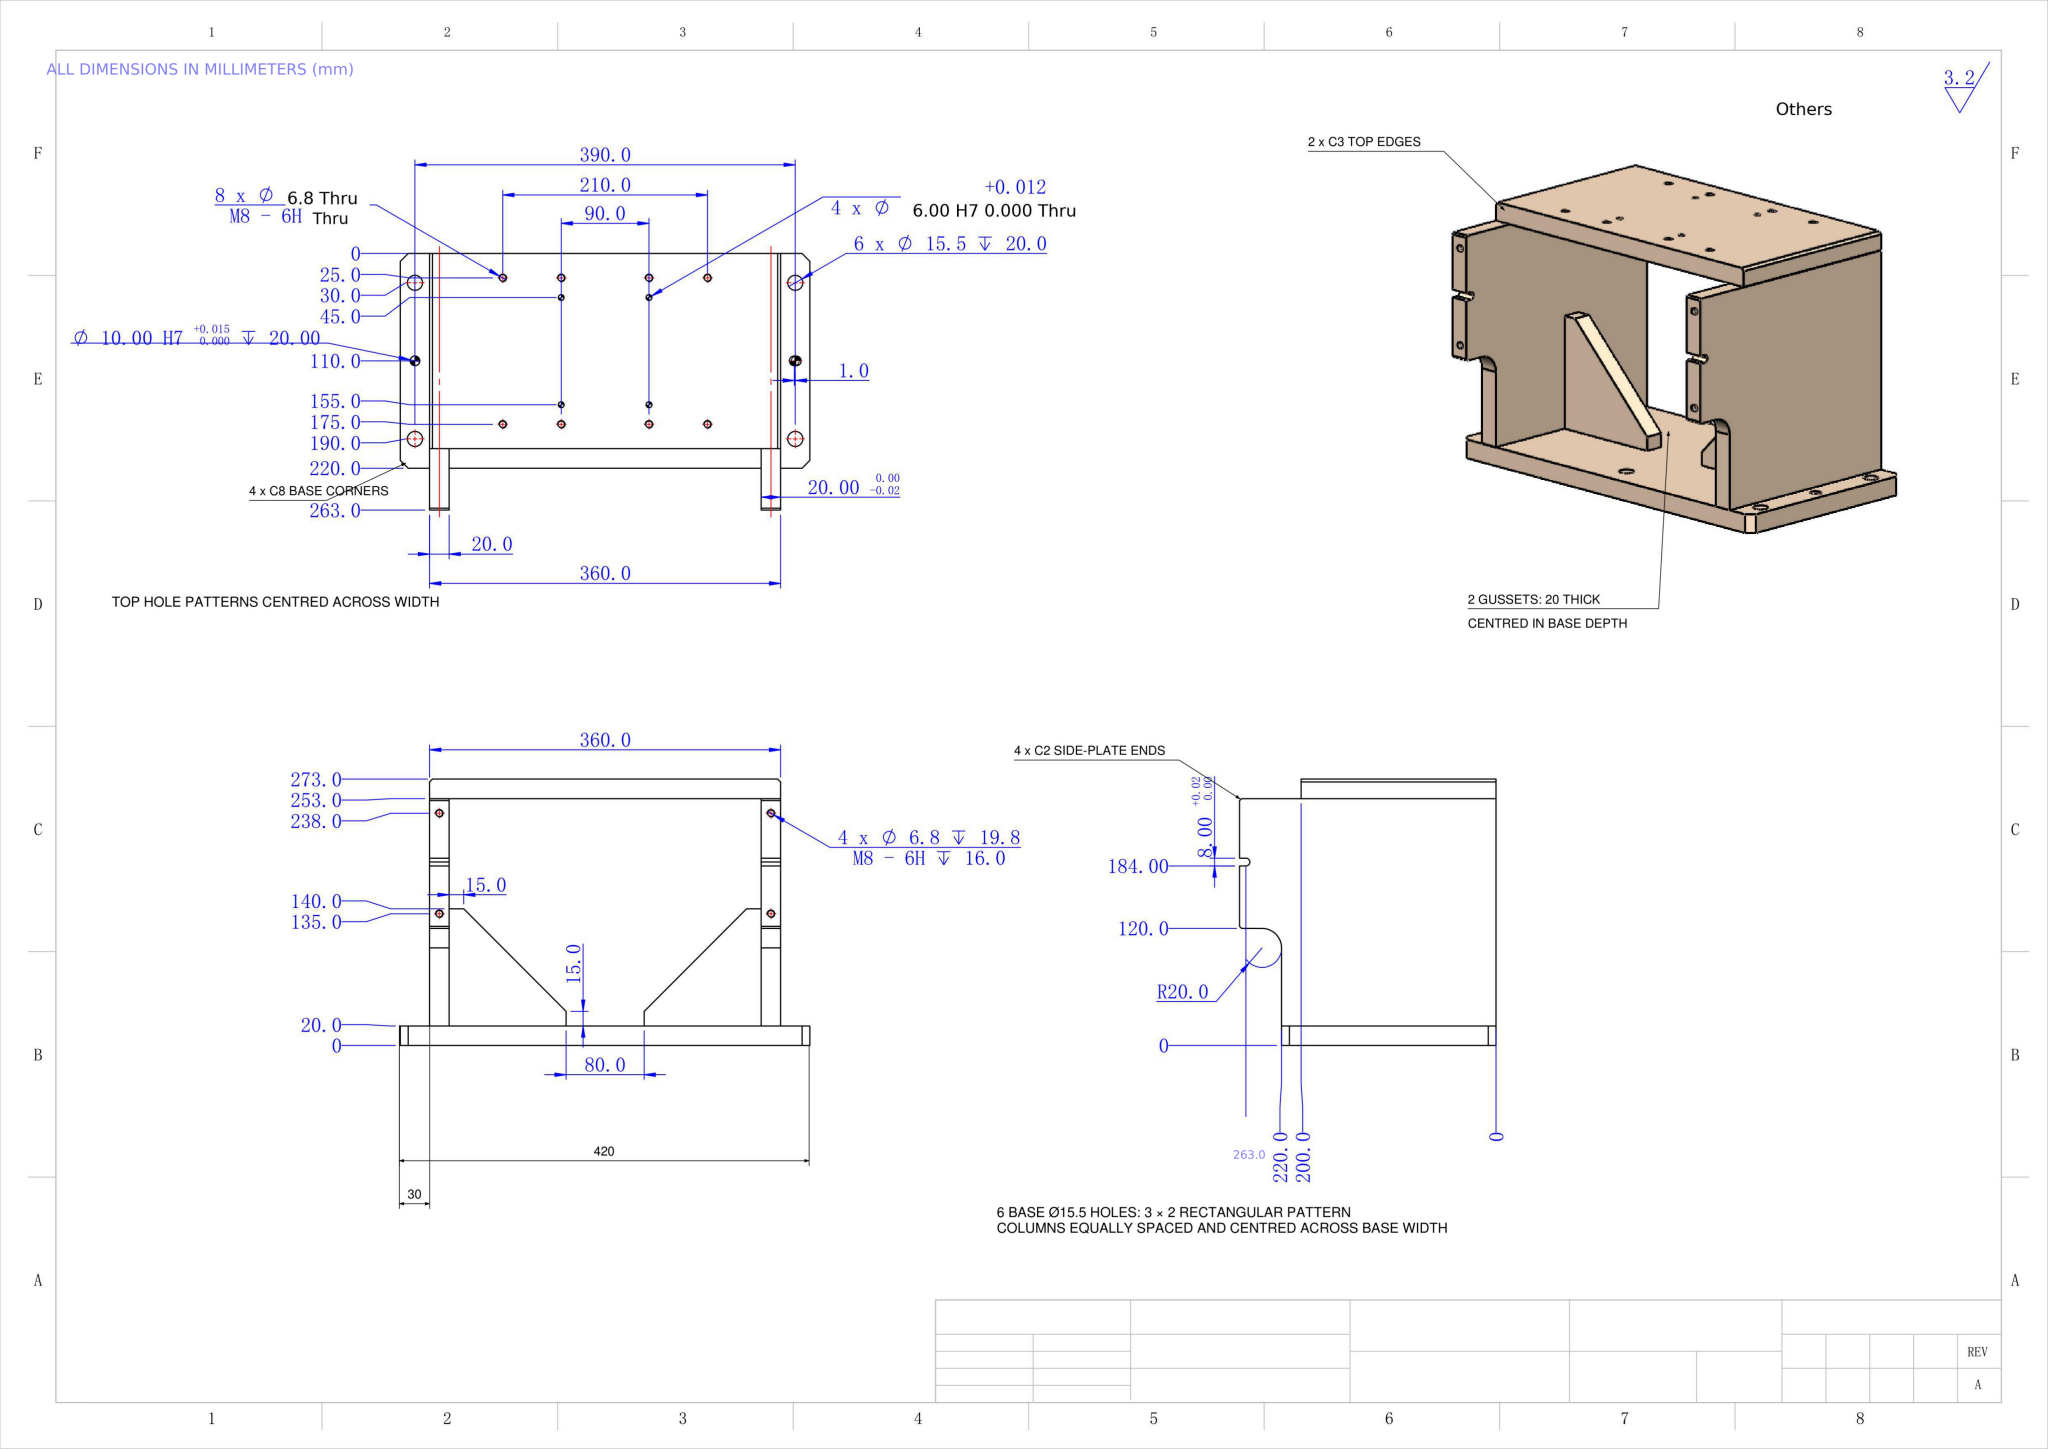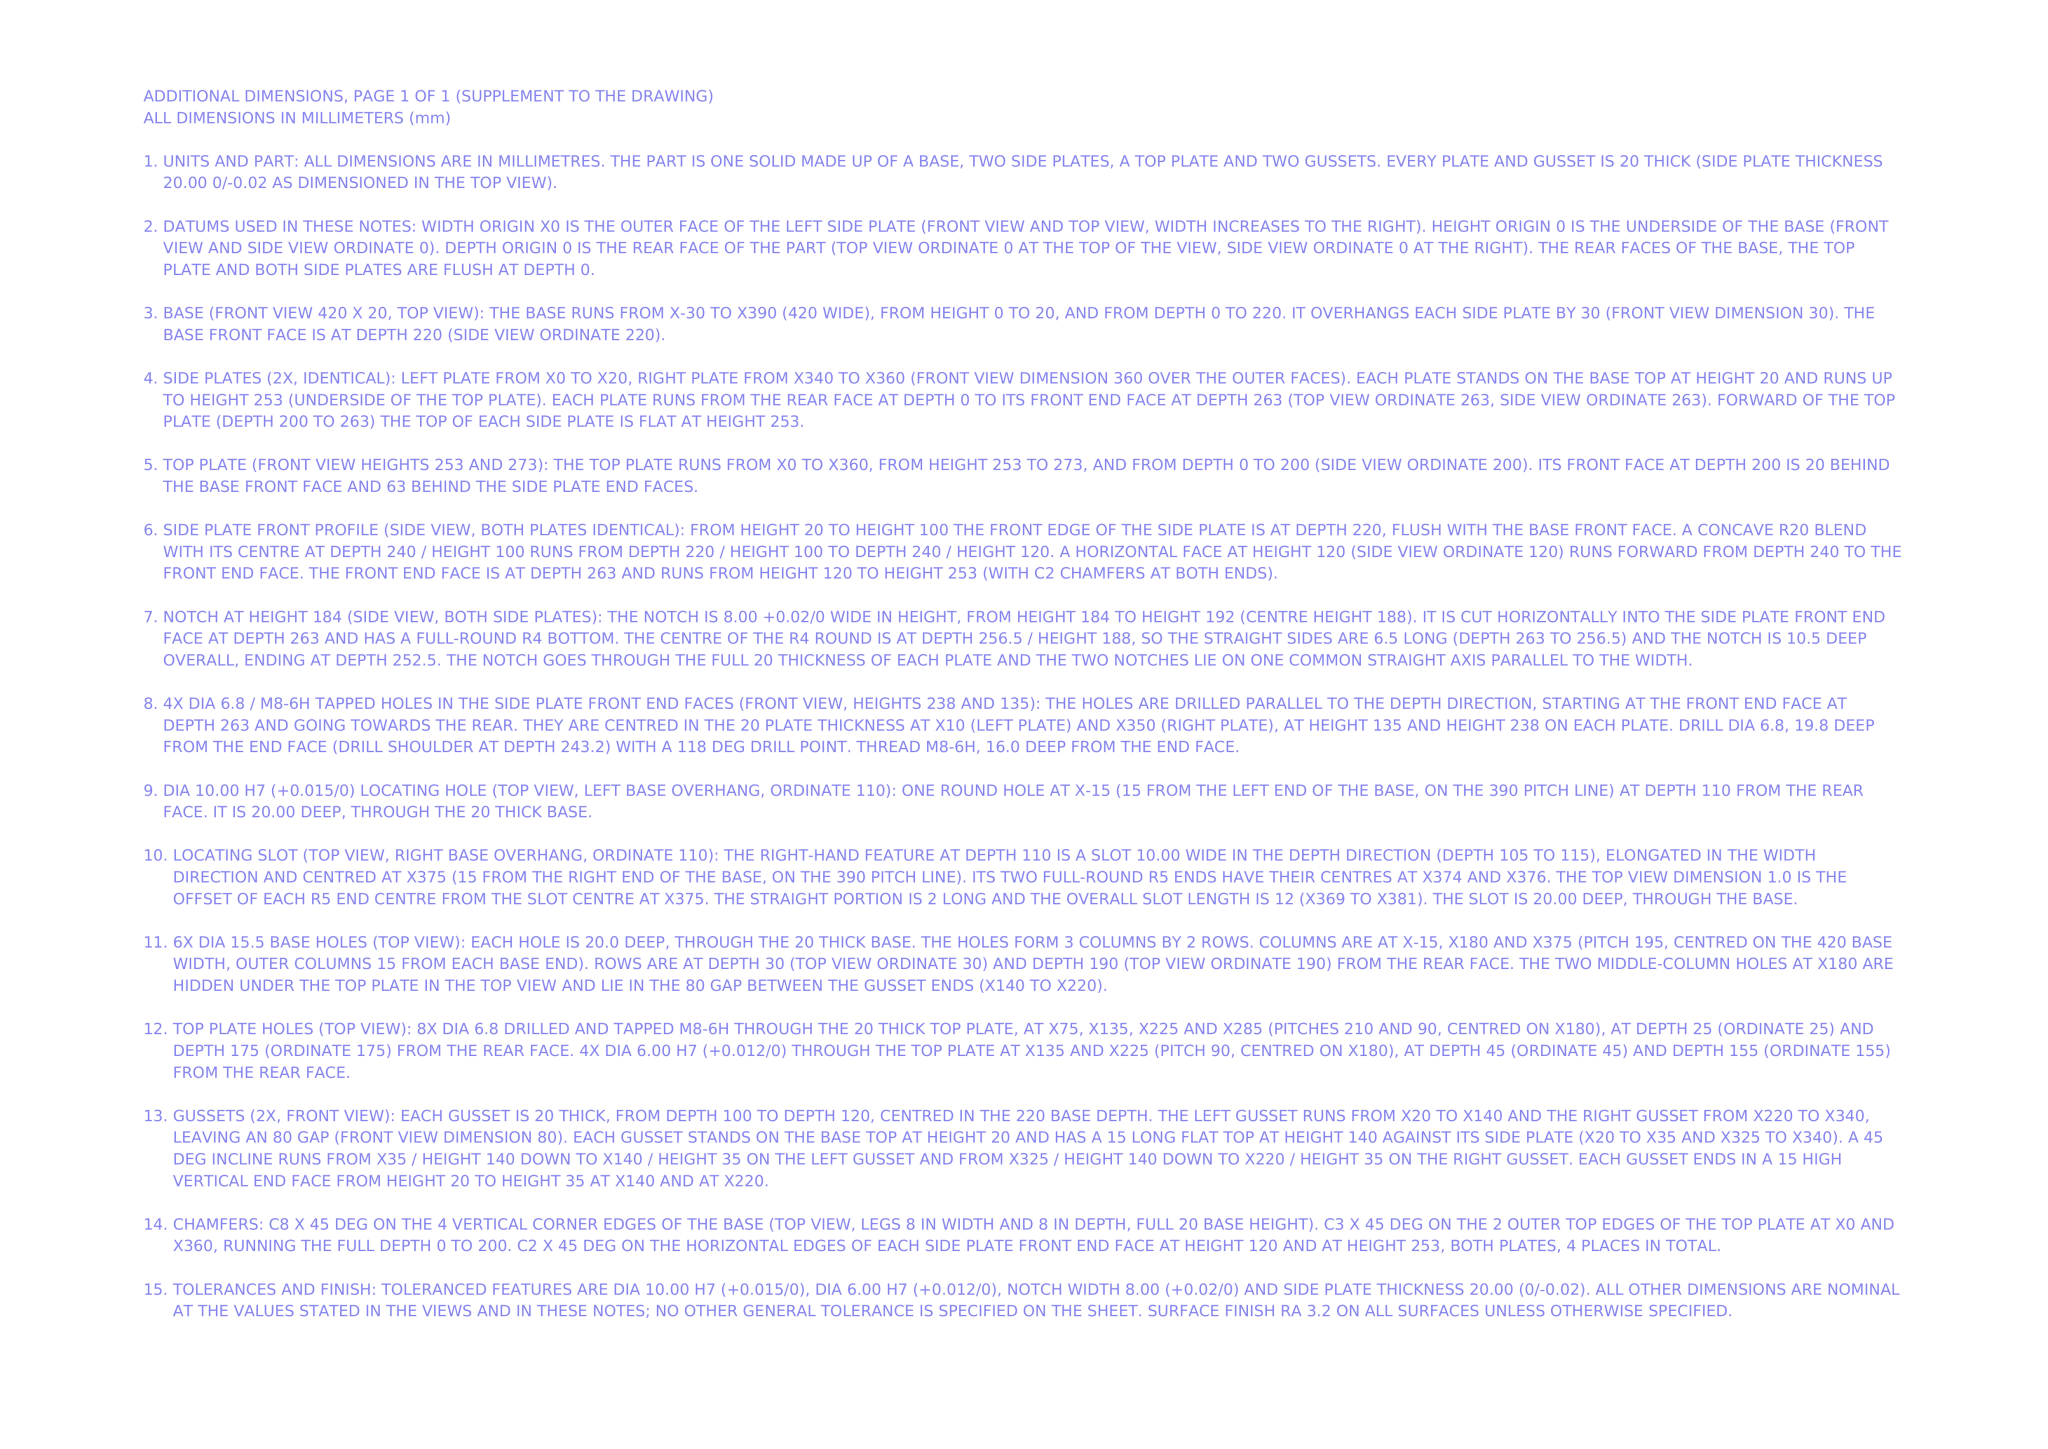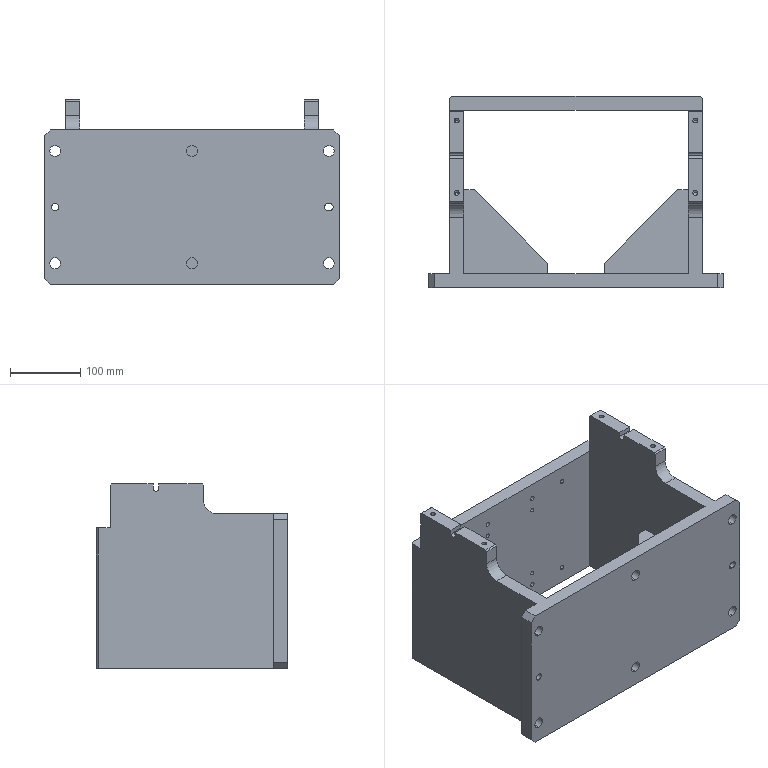Part | NX | mm | 1 solid | 111 faces | box 420 x 273 x 263 mm | volume 5881263 mm3 | cylinder 54 | plane 49 | cone 8 | commonest cylinder face diameters 6.8 x24 15.5 x12 6 x8 10 x4 8 x4 40 x2